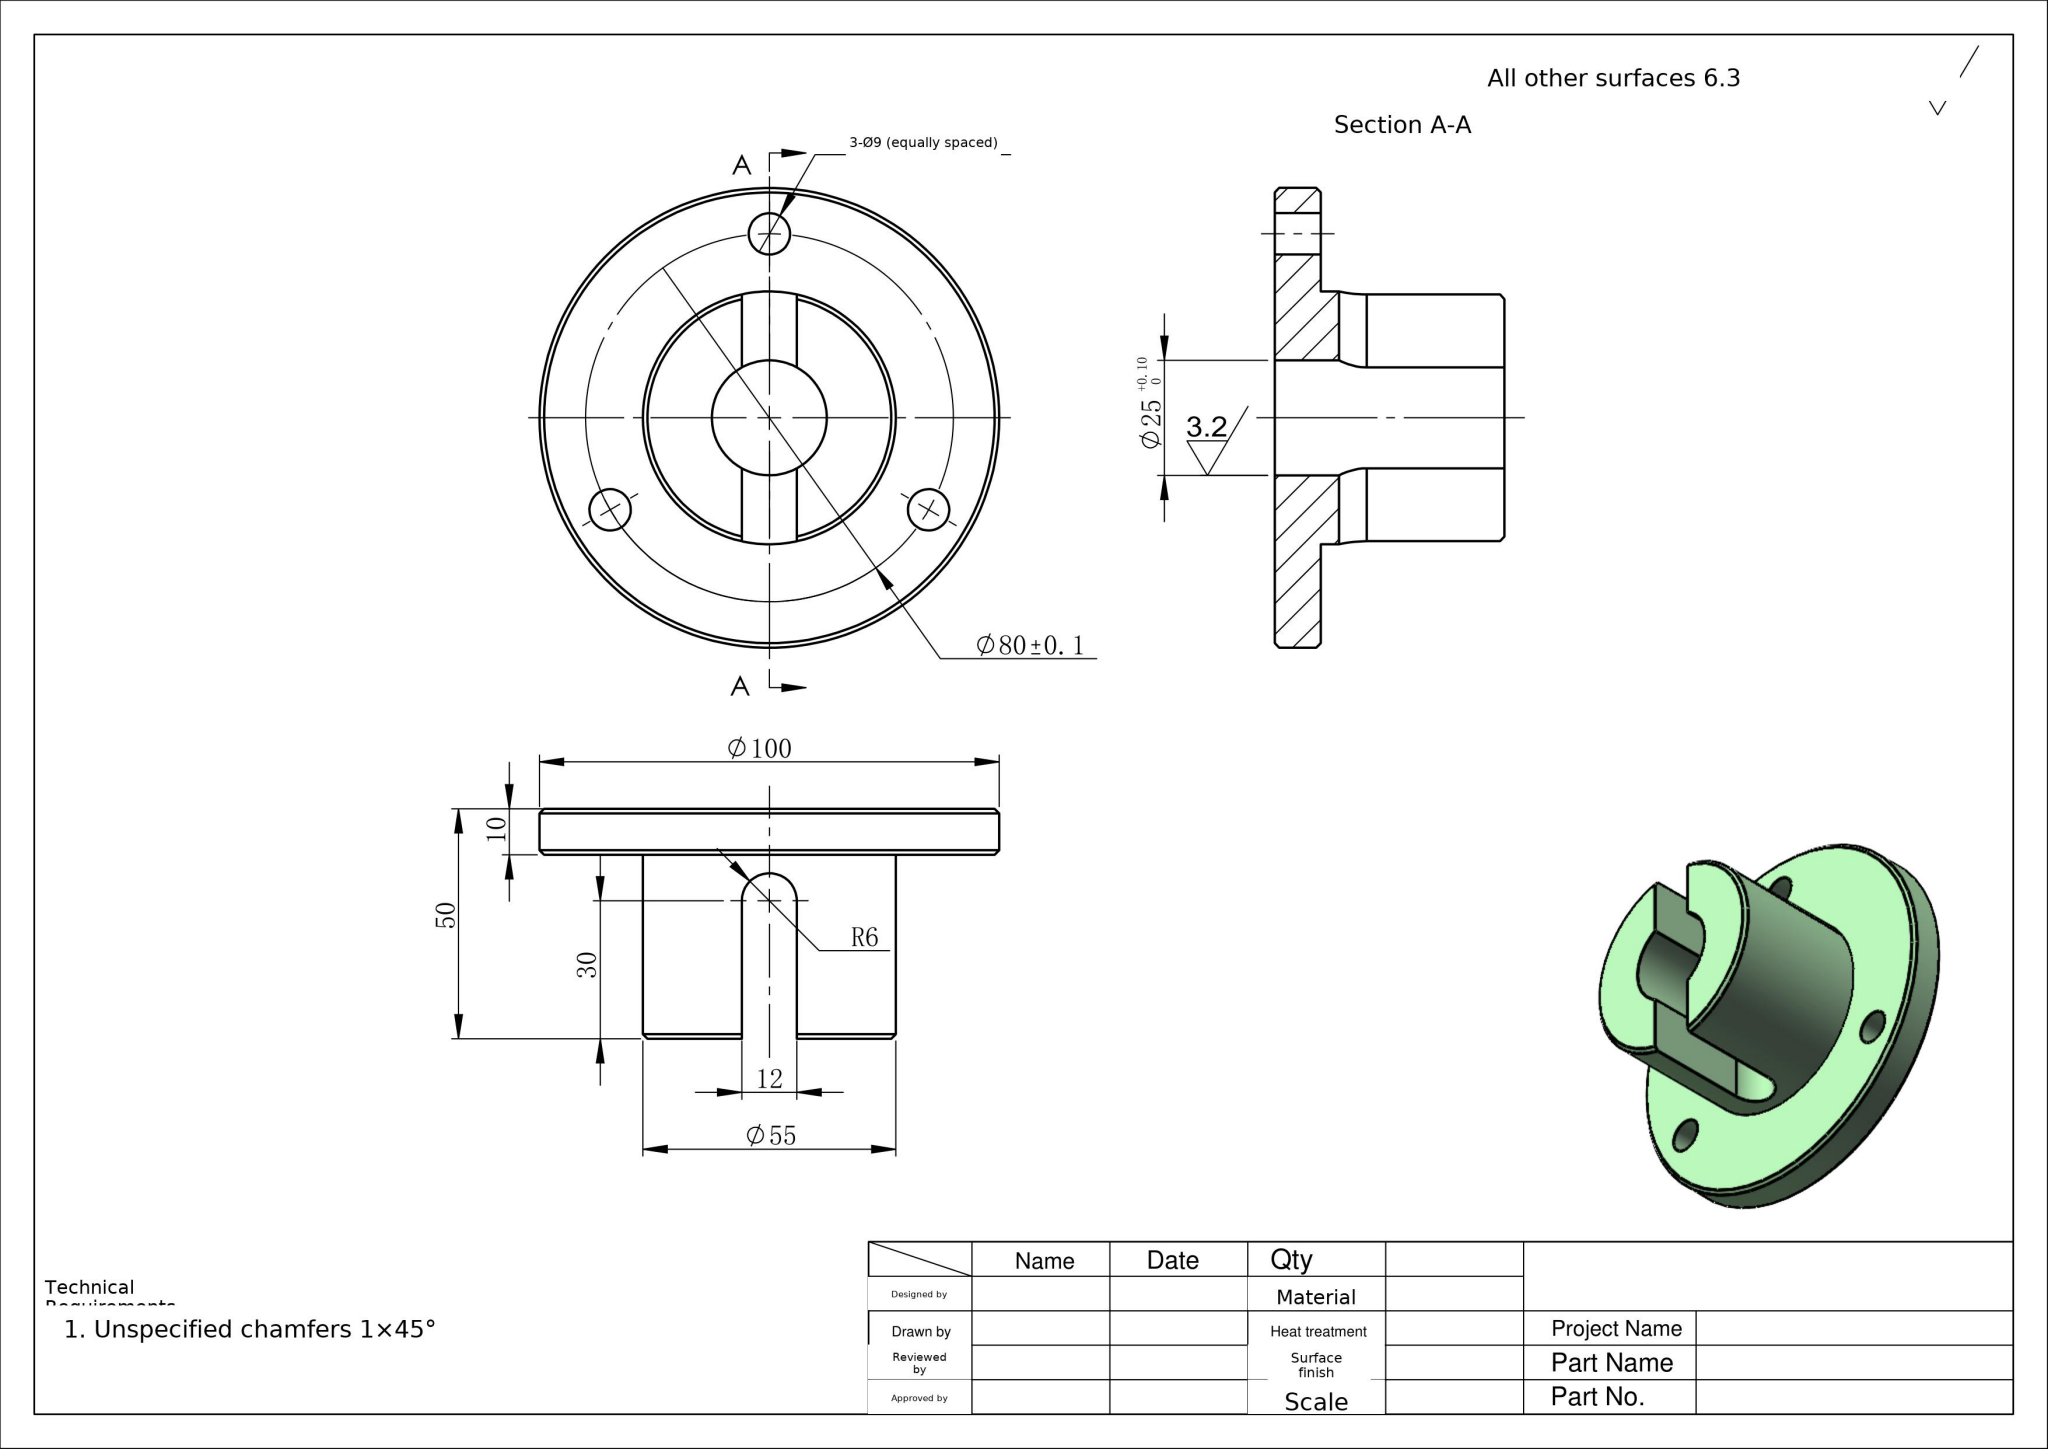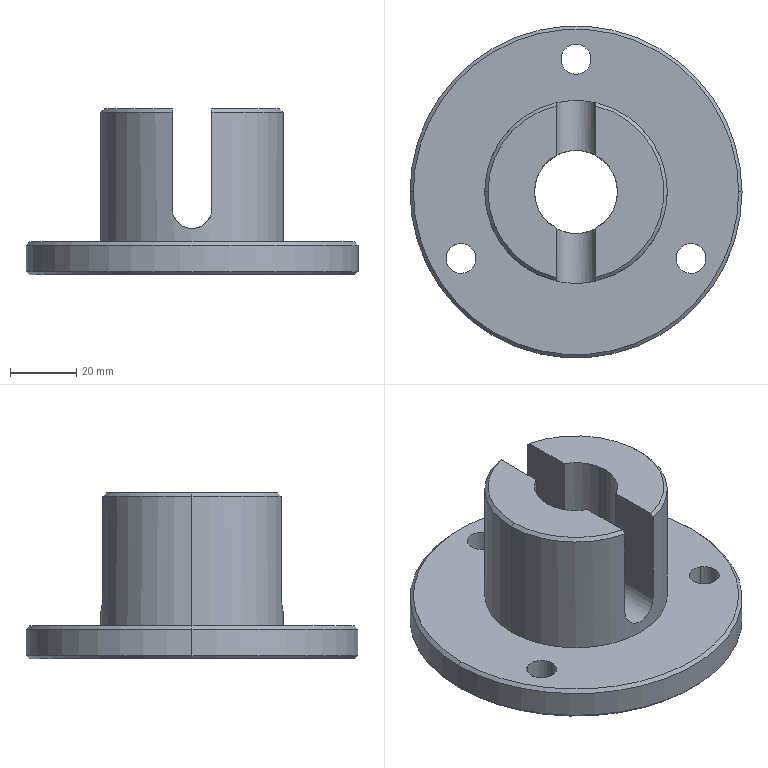Part | SolidWorks | mm | 1 solid | 29 faces | box 100 x 100 x 50 mm | volume 134015 mm3 | cylinder 14 | plane 8 | cone 7 | commonest cylinder face diameters 9 x6 100 x2 25 x2 55 x2 12 x2
build123d program:
from build123d import *

# Parameters (mm, degrees)
SKETCH1_R          = 27.5
SKETCH1_R_2        = 12.5
EXTRUDE1_DEPTH     = 50
SKETCH2_R          = 50
SKETCH2_R_2        = 27.5
EXTRUDE2_DEPTH     = 10
CUT_EXTRUDE1_DEPTH = 105.911
CHAMFER1_SIZE      = 1
SKETCH7_R          = 4.5
CUT_EXTRUDE4_DEPTH = 87.603
CIRPATTERN1_COUNT  = 3


with BuildPart() as part:
    # Sketch1 → Extrude1 (new body)
    with BuildSketch(Plane.XY):
        Circle(SKETCH1_R)
        Circle(SKETCH1_R_2, mode=Mode.SUBTRACT)
    extrude(amount=EXTRUDE1_DEPTH)

    # Sketch2 → Extrude2 (add)
    with BuildSketch(Plane(origin=(0, 0, 0), x_dir=(-1, 0, 0), z_dir=(0, 0, -1))):
        Circle(SKETCH2_R)
        Circle(SKETCH2_R_2, mode=Mode.SUBTRACT)
    extrude(amount=-EXTRUDE2_DEPTH)

    # Sketch4 → Cut-Extrude1 (cut, through all)
    with BuildSketch(Plane(origin=(0, 27.5, 0), x_dir=(-1, 0, 0), z_dir=(0, 1, 0))):
        with BuildLine():
            Line((-6, 20), (-6, 79.58))
            Line((-6, 79.58), (6, 79.58))
            Line((6, 79.58), (6, 20))
            ThreePointArc((6, 20), (0, 14), (-6, 20))
        make_face()
    extrude(amount=-CUT_EXTRUDE1_DEPTH, mode=Mode.SUBTRACT)

    # Chamfer1
    chamfer1_edges = [part.edges().sort_by_distance(p)[0] for p in [
        (50, 0, 10),
        (50, 0, 0),
        (-27.5, 0, 50),
        (21.462, 17.194, 50),
    ]]
    chamfer(chamfer1_edges, length=CHAMFER1_SIZE)

    # Sketch7 → Cut-Extrude4 (cut, through all)
    with BuildSketch(Plane(origin=(0, 0, 0), x_dir=(-1, 0, 0), z_dir=(0, 0, -1))):
        with Locations((0, 40)):
            Circle(SKETCH7_R)
    cut_extrude4 = extrude(amount=-CUT_EXTRUDE4_DEPTH, mode=Mode.SUBTRACT)

    # CirPattern1: Cut-Extrude4 ×3 about axis
    cirpattern1_axis = Axis((0, 0, 0), (0, 0, 1))
    for i in range(1, CIRPATTERN1_COUNT):
        add(cut_extrude4.rotate(cirpattern1_axis, i * 360 / CIRPATTERN1_COUNT), mode=Mode.SUBTRACT)


solid = part.part